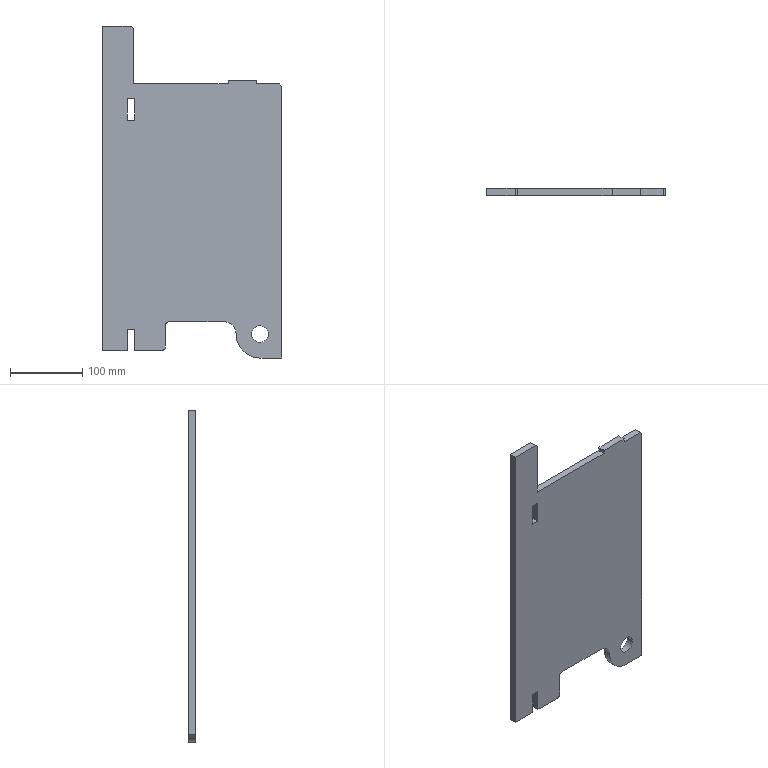Component | SolidWorks | RearUprightPlate-1 | 1 solid | 34 faces | box 247.5 x 10 x 458 mm | volume 902265 mm3 | plane 27 | cylinder 7 | commonest cylinder face diameters 23.2 x2 33.314 x2 10 x2 66 x1 | material Q235
build123d program:
from build123d import *

# Parameters (mm, degrees)
SKETCH1_R           = 11.6
BOSS_EXTRUDE1_DEPTH = 10


with BuildPart() as part:
    # Sketch1 → Boss-Extrude1 (new body)
    with BuildSketch(Plane.XY):
        with BuildLine():
            Line((3719.424, 1887.781), (3719.424, 1862.781))
            Line((3719.424, 1862.781), (3719.424, 1857.781))
            ThreePointArc((3719.424, 1857.781), (3720.888, 1854.245), (3724.424, 1852.781))
            Line((3724.424, 1852.781), (3754.824, 1852.781))
            Line((3754.824, 1852.781), (3755.824, 1852.781))
            Line((3755.824, 1852.781), (3758.924, 1852.781))
            Line((3758.924, 1852.781), (3761.824, 1852.781))
            Line((3761.824, 1852.781), (3761.824, 1882.781))
            Line((3761.824, 1882.781), (3772.024, 1882.781))
            Line((3772.024, 1882.781), (3772.024, 1852.781))
            Line((3772.024, 1852.781), (3774.824, 1852.781))
            Line((3774.824, 1852.781), (3806.424, 1852.781))
            Line((3806.424, 1852.781), (3806.424, 2300.781))
            Line((3806.424, 2300.781), (3766.424, 2300.781))
            Line((3766.424, 2300.781), (3763.424, 2297.781))
            Line((3763.424, 2297.781), (3763.424, 2250.781))
            Line((3763.424, 2250.781), (3763.424, 2220.781))
            Line((3763.424, 2220.781), (3632.924, 2220.781))
            Line((3632.924, 2220.781), (3632.924, 2225.781))
            Line((3632.924, 2225.781), (3593.924, 2225.781))
            Line((3593.924, 2225.781), (3593.924, 2220.781))
            Line((3593.924, 2220.781), (3561.924, 2220.781))
            Line((3561.924, 2220.781), (3558.924, 2217.781))
            Line((3558.924, 2217.781), (3558.924, 1842.781))
            Line((3558.924, 1842.781), (3577.54, 1842.781))
            Line((3577.54, 1842.781), (3588.924, 1842.781))
            ThreePointArc((3588.924, 1842.781), (3612.258, 1852.446), (3621.924, 1875.781))
            ThreePointArc((3621.924, 1875.781), (3626.519, 1887.627), (3638.131, 1892.787))
            Line((3638.131, 1892.787), (3713.924, 1892.781))
            Line((3713.924, 1892.781), (3714.424, 1892.781))
            ThreePointArc((3714.424, 1892.781), (3717.959, 1891.316), (3719.424, 1887.781))
        make_face()
        with Locations((3588.924, 1875.781)):
            Circle(SKETCH1_R, mode=Mode.SUBTRACT)
        Polygon((3772.024, 2170.781), (3761.824, 2170.781), (3761.824, 2200.781), (3772.024, 2200.781), (3772.024, 2190.781), align=None, mode=Mode.SUBTRACT)
    extrude(amount=BOSS_EXTRUDE1_DEPTH)


solid = part.part

# Placed as in the assembly
solid = solid.moved(Location((3301.77, -165.326, 514.924), (-90, 0, 180)))
STEP:
#1=CARTESIAN_POINT('',(-10.849,-6.115,94.122));
#2=VERTEX_POINT('',#1);
#3=CARTESIAN_POINT('',(-11.762,-6.115,94.122));
#4=VERTEX_POINT('',#3);
#5=CARTESIAN_POINT('',(-11.305,-6.115,94.122));
#6=DIRECTION('',(-0.,1.,-0.));
#7=DIRECTION('',(-1.,0.,0.));
#8=AXIS2_PLACEMENT_3D('',#5,#6,#7);
#9=CIRCLE('',#8,0.4567);
#10=EDGE_CURVE('',#2,#4,#9,.T.);
#11=ORIENTED_EDGE('',*,*,#10,.T.);
#12=CARTESIAN_POINT('',(-11.762,-6.509,94.122));
#13=VERTEX_POINT('',#12);
#14=CARTESIAN_POINT('',(-11.762,-6.115,94.122));
#15=DIRECTION('',(0.,-1.,0.));
#16=VECTOR('',#15,39.37);
#17=LINE('',#14,#16);
#18=EDGE_CURVE('',#4,#13,#17,.T.);
#19=ORIENTED_EDGE('',*,*,#18,.T.);
#20=CARTESIAN_POINT('',(-10.849,-6.509,94.122));
#21=VERTEX_POINT('',#20);
#22=CARTESIAN_POINT('',(-11.305,-6.509,94.122));
#23=DIRECTION('',(-0.,1.,-0.));
#24=DIRECTION('',(-1.,0.,0.));
#25=AXIS2_PLACEMENT_3D('',#22,#23,#24);
#26=CIRCLE('',#25,0.4567);
#27=EDGE_CURVE('',#21,#13,#26,.T.);
#28=ORIENTED_EDGE('',*,*,#27,.F.);
#29=CARTESIAN_POINT('',(-10.849,-6.115,94.122));
#30=DIRECTION('',(0.,-1.,0.));
#31=VECTOR('',#30,39.37);
#32=LINE('',#29,#31);
#33=EDGE_CURVE('',#2,#21,#32,.T.);
#34=ORIENTED_EDGE('',*,*,#33,.F.);
#35=EDGE_LOOP('',(#11,#19,#28,#34));
#36=FACE_OUTER_BOUND('',#35,.T.);
#37=CARTESIAN_POINT('',(-11.305,-6.115,94.122));
#38=DIRECTION('',(0.,-1.,0.));
#39=DIRECTION('',(1.,0.,0.));
#40=AXIS2_PLACEMENT_3D('',#37,#38,#39);
#41=CYLINDRICAL_SURFACE('',#40,0.4567);
#42=ADVANCED_FACE('',(#36),#41,.F.);
#43=CARTESIAN_POINT('',(-13.243,-6.115,94.792));
#44=VERTEX_POINT('',#43);
#45=CARTESIAN_POINT('',(-12.604,-6.115,94.136));
#46=VERTEX_POINT('',#45);
#47=CARTESIAN_POINT('',(-13.26,-6.115,94.136));
#48=DIRECTION('',(-0.,1.,-0.));
#49=DIRECTION('',(-1.,0.,0.));
#50=AXIS2_PLACEMENT_3D('',#47,#48,#49);
#51=CIRCLE('',#50,0.6558);
#52=EDGE_CURVE('',#44,#46,#51,.T.);
#53=ORIENTED_EDGE('',*,*,#52,.T.);
#54=CARTESIAN_POINT('',(-12.604,-6.509,94.136));
#55=VERTEX_POINT('',#54);
#56=CARTESIAN_POINT('',(-12.604,-6.115,94.136));
#57=DIRECTION('',(0.,-1.,0.));
#58=VECTOR('',#57,39.37);
#59=LINE('',#56,#58);
#60=EDGE_CURVE('',#46,#55,#59,.T.);
#61=ORIENTED_EDGE('',*,*,#60,.T.);
#62=CARTESIAN_POINT('',(-13.243,-6.509,94.792));
#63=VERTEX_POINT('',#62);
#64=CARTESIAN_POINT('',(-13.26,-6.509,94.136));
#65=DIRECTION('',(-0.,1.,-0.));
#66=DIRECTION('',(-1.,0.,0.));
#67=AXIS2_PLACEMENT_3D('',#64,#65,#66);
#68=CIRCLE('',#67,0.6558);
#69=EDGE_CURVE('',#63,#55,#68,.T.);
#70=ORIENTED_EDGE('',*,*,#69,.F.);
#71=CARTESIAN_POINT('',(-13.243,-6.115,94.792));
#72=DIRECTION('',(0.,-1.,0.));
#73=VECTOR('',#72,39.37);
#74=LINE('',#71,#73);
#75=EDGE_CURVE('',#44,#63,#74,.T.);
#76=ORIENTED_EDGE('',*,*,#75,.F.);
#77=EDGE_LOOP('',(#53,#61,#70,#76));
#78=FACE_OUTER_BOUND('',#77,.T.);
#79=CARTESIAN_POINT('',(-13.26,-6.115,94.136));
#80=DIRECTION('',(0.,-1.,0.));
#81=DIRECTION('',(1.,0.,0.));
#82=AXIS2_PLACEMENT_3D('',#79,#80,#81);
#83=CYLINDRICAL_SURFACE('',#82,0.6558);
#84=ADVANCED_FACE('',(#78),#83,.F.);
#85=CARTESIAN_POINT('',(-11.305,-6.509,92.823));
#86=VERTEX_POINT('',#85);
#87=CARTESIAN_POINT('',(-10.124,-6.509,92.823));
#88=VERTEX_POINT('',#87);
#89=CARTESIAN_POINT('',(129.991,-6.509,92.823));
#90=DIRECTION('',(1.,0.,0.));
#91=VECTOR('',#90,39.37);
#92=LINE('',#89,#91);
#93=EDGE_CURVE('',#86,#88,#92,.T.);
#94=ORIENTED_EDGE('',*,*,#93,.F.);
#95=CARTESIAN_POINT('',(-11.305,-6.115,92.823));
#96=VERTEX_POINT('',#95);
#97=CARTESIAN_POINT('',(-11.305,-6.115,92.823));
#98=DIRECTION('',(0.,-1.,0.));
#99=VECTOR('',#98,39.37);
#100=LINE('',#97,#99);
#101=EDGE_CURVE('',#96,#86,#100,.T.);
#102=ORIENTED_EDGE('',*,*,#101,.F.);
#103=CARTESIAN_POINT('',(-10.124,-6.115,92.823));
#104=VERTEX_POINT('',#103);
#105=CARTESIAN_POINT('',(129.991,-6.115,92.823));
#106=DIRECTION('',(1.,0.,0.));
#107=VECTOR('',#106,39.37);
#108=LINE('',#105,#107);
#109=EDGE_CURVE('',#96,#104,#108,.T.);
#110=ORIENTED_EDGE('',*,*,#109,.T.);
#111=CARTESIAN_POINT('',(-10.124,-6.115,92.823));
#112=DIRECTION('',(0.,-1.,0.));
#113=VECTOR('',#112,39.37);
#114=LINE('',#111,#113);
#115=EDGE_CURVE('',#104,#88,#114,.T.);
#116=ORIENTED_EDGE('',*,*,#115,.T.);
#117=EDGE_LOOP('',(#94,#102,#110,#116));
#118=FACE_OUTER_BOUND('',#117,.T.);
#119=CARTESIAN_POINT('',(129.991,-6.115,92.823));
#120=DIRECTION('',(0.,-0.,-1.));
#121=DIRECTION('',(0.,-1.,0.));
#122=AXIS2_PLACEMENT_3D('',#119,#120,#121);
#123=PLANE('',#122);
#124=ADVANCED_FACE('',(#118),#123,.T.);
#125=CARTESIAN_POINT('',(-12.604,-6.509,94.122));
#126=VERTEX_POINT('',#125);
#127=CARTESIAN_POINT('',(-11.305,-6.509,94.122));
#128=DIRECTION('',(-0.,1.,-0.));
#129=DIRECTION('',(-1.,0.,0.));
#130=AXIS2_PLACEMENT_3D('',#127,#128,#129);
#131=CIRCLE('',#130,1.299);
#132=EDGE_CURVE('',#86,#126,#131,.T.);
#133=ORIENTED_EDGE('',*,*,#132,.T.);
#134=CARTESIAN_POINT('',(-12.604,-6.115,94.122));
#135=VERTEX_POINT('',#134);
#136=CARTESIAN_POINT('',(-12.604,-6.115,94.122));
#137=DIRECTION('',(0.,-1.,0.));
#138=VECTOR('',#137,39.37);
#139=LINE('',#136,#138);
#140=EDGE_CURVE('',#135,#126,#139,.T.);
#141=ORIENTED_EDGE('',*,*,#140,.F.);
#142=CARTESIAN_POINT('',(-11.305,-6.115,94.122));
#143=DIRECTION('',(-0.,1.,-0.));
#144=DIRECTION('',(-1.,0.,0.));
#145=AXIS2_PLACEMENT_3D('',#142,#143,#144);
#146=CIRCLE('',#145,1.299);
#147=EDGE_CURVE('',#96,#135,#146,.T.);
#148=ORIENTED_EDGE('',*,*,#147,.F.);
#149=ORIENTED_EDGE('',*,*,#101,.T.);
#150=EDGE_LOOP('',(#133,#141,#148,#149));
#151=FACE_OUTER_BOUND('',#150,.T.);
#152=CARTESIAN_POINT('',(-11.305,-6.115,94.122));
#153=DIRECTION('',(0.,-1.,0.));
#154=DIRECTION('',(1.,0.,0.));
#155=AXIS2_PLACEMENT_3D('',#152,#153,#154);
#156=CYLINDRICAL_SURFACE('',#155,1.299);
#157=ADVANCED_FACE('',(#151),#156,.T.);
#158=ORIENTED_EDGE('',*,*,#60,.F.);
#159=CARTESIAN_POINT('',(-13.26,-6.115,94.136));
#160=DIRECTION('',(-0.,1.,-0.));
#161=DIRECTION('',(-1.,0.,0.));
#162=AXIS2_PLACEMENT_3D('',#159,#160,#161);
#163=CIRCLE('',#162,0.6558);
#164=EDGE_CURVE('',#46,#135,#163,.T.);
#165=ORIENTED_EDGE('',*,*,#164,.T.);
#166=ORIENTED_EDGE('',*,*,#140,.T.);
#167=CARTESIAN_POINT('',(-13.26,-6.509,94.136));
#168=DIRECTION('',(-0.,1.,-0.));
#169=DIRECTION('',(-1.,0.,0.));
#170=AXIS2_PLACEMENT_3D('',#167,#168,#169);
#171=CIRCLE('',#170,0.6558);
#172=EDGE_CURVE('',#55,#126,#171,.T.);
#173=ORIENTED_EDGE('',*,*,#172,.F.);
#174=EDGE_LOOP('',(#158,#165,#166,#173));
#175=FACE_OUTER_BOUND('',#174,.T.);
#176=CARTESIAN_POINT('',(-13.26,-6.115,94.136));
#177=DIRECTION('',(0.,-1.,0.));
#178=DIRECTION('',(1.,0.,0.));
#179=AXIS2_PLACEMENT_3D('',#176,#177,#178);
#180=CYLINDRICAL_SURFACE('',#179,0.6558);
#181=ADVANCED_FACE('',(#175),#180,.F.);
#182=CARTESIAN_POINT('',(-16.227,-6.509,94.792));
#183=VERTEX_POINT('',#182);
#184=CARTESIAN_POINT('',(129.985,-6.509,94.803));
#185=DIRECTION('',(-1.,-0.,-0.00008077));
#186=VECTOR('',#185,39.37);
#187=LINE('',#184,#186);
#188=EDGE_CURVE('',#63,#183,#187,.T.);
#189=ORIENTED_EDGE('',*,*,#188,.T.);
#190=CARTESIAN_POINT('',(-16.227,-6.115,94.792));
#191=VERTEX_POINT('',#190);
#192=CARTESIAN_POINT('',(-16.227,-6.115,94.792));
#193=DIRECTION('',(0.,-1.,0.));
#194=VECTOR('',#193,39.37);
#195=LINE('',#192,#194);
#196=EDGE_CURVE('',#191,#183,#195,.T.);
#197=ORIENTED_EDGE('',*,*,#196,.F.);
#198=CARTESIAN_POINT('',(129.985,-6.115,94.803));
#199=DIRECTION('',(-1.,-0.,-0.00008077));
#200=VECTOR('',#199,39.37);
#201=LINE('',#198,#200);
#202=EDGE_CURVE('',#44,#191,#201,.T.);
#203=ORIENTED_EDGE('',*,*,#202,.F.);
#204=ORIENTED_EDGE('',*,*,#75,.T.);
#205=EDGE_LOOP('',(#189,#197,#203,#204));
#206=FACE_OUTER_BOUND('',#205,.T.);
#207=CARTESIAN_POINT('',(129.985,-6.115,94.803));
#208=DIRECTION('',(-0.00008077,0.,1.));
#209=DIRECTION('',(1.,0.,0.00008077));
#210=AXIS2_PLACEMENT_3D('',#207,#208,#209);
#211=PLANE('',#210);
#212=ADVANCED_FACE('',(#206),#211,.F.);
#213=CARTESIAN_POINT('',(-16.246,-6.509,94.792));
#214=VERTEX_POINT('',#213);
#215=CARTESIAN_POINT('',(129.991,-6.509,94.792));
#216=DIRECTION('',(-1.,-0.,-0.));
#217=VECTOR('',#216,39.37);
#218=LINE('',#215,#217);
#219=EDGE_CURVE('',#183,#214,#218,.T.);
#220=ORIENTED_EDGE('',*,*,#219,.T.);
#221=CARTESIAN_POINT('',(-16.246,-6.115,94.792));
#222=VERTEX_POINT('',#221);
#223=CARTESIAN_POINT('',(-16.246,-6.115,94.792));
#224=DIRECTION('',(0.,-1.,0.));
#225=VECTOR('',#224,39.37);
#226=LINE('',#223,#225);
#227=EDGE_CURVE('',#222,#214,#226,.T.);
#228=ORIENTED_EDGE('',*,*,#227,.F.);
#229=CARTESIAN_POINT('',(129.991,-6.115,94.792));
#230=DIRECTION('',(-1.,-0.,-0.));
#231=VECTOR('',#230,39.37);
#232=LINE('',#229,#231);
#233=EDGE_CURVE('',#191,#222,#232,.T.);
#234=ORIENTED_EDGE('',*,*,#233,.F.);
#235=ORIENTED_EDGE('',*,*,#196,.T.);
#236=EDGE_LOOP('',(#220,#228,#234,#235));
#237=FACE_OUTER_BOUND('',#236,.T.);
#238=CARTESIAN_POINT('',(129.991,-6.115,94.792));
#239=DIRECTION('',(-0.,0.,1.));
#240=DIRECTION('',(-0.,1.,-0.));
#241=AXIS2_PLACEMENT_3D('',#238,#239,#240);
#242=PLANE('',#241);
#243=ADVANCED_FACE('',(#237),#242,.F.);
#244=CARTESIAN_POINT('',(-16.443,-6.509,94.595));
#245=VERTEX_POINT('',#244);
#246=CARTESIAN_POINT('',(-16.246,-6.509,94.595));
#247=DIRECTION('',(-0.,1.,-0.));
#248=DIRECTION('',(-1.,0.,0.));
#249=AXIS2_PLACEMENT_3D('',#246,#247,#248);
#250=CIRCLE('',#249,0.1969);
#251=EDGE_CURVE('',#245,#214,#250,.T.);
#252=ORIENTED_EDGE('',*,*,#251,.F.);
#253=CARTESIAN_POINT('',(-16.443,-6.115,94.595));
#254=VERTEX_POINT('',#253);
#255=CARTESIAN_POINT('',(-16.443,-6.115,94.595));
#256=DIRECTION('',(0.,-1.,0.));
#257=VECTOR('',#256,39.37);
#258=LINE('',#255,#257);
#259=EDGE_CURVE('',#254,#245,#258,.T.);
#260=ORIENTED_EDGE('',*,*,#259,.F.);
#261=CARTESIAN_POINT('',(-16.246,-6.115,94.595));
#262=DIRECTION('',(-0.,1.,-0.));
#263=DIRECTION('',(-1.,0.,0.));
#264=AXIS2_PLACEMENT_3D('',#261,#262,#263);
#265=CIRCLE('',#264,0.1969);
#266=EDGE_CURVE('',#254,#222,#265,.T.);
#267=ORIENTED_EDGE('',*,*,#266,.T.);
#268=ORIENTED_EDGE('',*,*,#227,.T.);
#269=EDGE_LOOP('',(#252,#260,#267,#268));
#270=FACE_OUTER_BOUND('',#269,.T.);
#271=CARTESIAN_POINT('',(-16.246,-6.115,94.595));
#272=DIRECTION('',(0.,-1.,0.));
#273=DIRECTION('',(1.,0.,0.));
#274=AXIS2_PLACEMENT_3D('',#271,#272,#273);
#275=CYLINDRICAL_SURFACE('',#274,0.1969);
#276=ADVANCED_FACE('',(#270),#275,.F.);
#277=CARTESIAN_POINT('',(-16.443,-6.509,93.61));
#278=VERTEX_POINT('',#277);
#279=CARTESIAN_POINT('',(-16.443,-6.509,20.273));
#280=DIRECTION('',(-0.00000029,0.,1.));
#281=VECTOR('',#280,39.37);
#282=LINE('',#279,#281);
#283=EDGE_CURVE('',#278,#245,#282,.T.);
#284=ORIENTED_EDGE('',*,*,#283,.F.);
#285=CARTESIAN_POINT('',(-16.443,-6.115,93.61));
#286=VERTEX_POINT('',#285);
#287=CARTESIAN_POINT('',(-16.443,-6.115,93.61));
#288=DIRECTION('',(0.,-1.,0.));
#289=VECTOR('',#288,39.37);
#290=LINE('',#287,#289);
#291=EDGE_CURVE('',#286,#278,#290,.T.);
#292=ORIENTED_EDGE('',*,*,#291,.F.);
#293=CARTESIAN_POINT('',(-16.443,-6.115,20.273));
#294=DIRECTION('',(-0.00000029,0.,1.));
#295=VECTOR('',#294,39.37);
#296=LINE('',#293,#295);
#297=EDGE_CURVE('',#286,#254,#296,.T.);
#298=ORIENTED_EDGE('',*,*,#297,.T.);
#299=ORIENTED_EDGE('',*,*,#259,.T.);
#300=EDGE_LOOP('',(#284,#292,#298,#299));
#301=FACE_OUTER_BOUND('',#300,.T.);
#302=CARTESIAN_POINT('',(-16.443,-6.115,20.273));
#303=DIRECTION('',(1.,0.,0.00000029));
#304=DIRECTION('',(0.00000029,-0.,-1.));
#305=AXIS2_PLACEMENT_3D('',#302,#303,#304);
#306=PLANE('',#305);
#307=ADVANCED_FACE('',(#301),#306,.T.);
#308=CARTESIAN_POINT('',(-16.443,-6.509,93.414));
#309=VERTEX_POINT('',#308);
#310=CARTESIAN_POINT('',(-16.443,-6.509,20.273));
#311=DIRECTION('',(-0.00000143,-0.,-1.));
#312=VECTOR('',#311,39.37);
#313=LINE('',#310,#312);
#314=EDGE_CURVE('',#278,#309,#313,.T.);
#315=ORIENTED_EDGE('',*,*,#314,.T.);
#316=CARTESIAN_POINT('',(-16.443,-6.115,93.414));
#317=VERTEX_POINT('',#316);
#318=CARTESIAN_POINT('',(-16.443,-6.115,93.414));
#319=DIRECTION('',(0.,-1.,0.));
#320=VECTOR('',#319,39.37);
#321=LINE('',#318,#320);
#322=EDGE_CURVE('',#317,#309,#321,.T.);
#323=ORIENTED_EDGE('',*,*,#322,.F.);
#324=CARTESIAN_POINT('',(-16.443,-6.115,20.273));
#325=DIRECTION('',(-0.00000143,-0.,-1.));
#326=VECTOR('',#325,39.37);
#327=LINE('',#324,#326);
#328=EDGE_CURVE('',#286,#317,#327,.T.);
#329=ORIENTED_EDGE('',*,*,#328,.F.);
#330=ORIENTED_EDGE('',*,*,#291,.T.);
#331=EDGE_LOOP('',(#315,#323,#329,#330));
#332=FACE_OUTER_BOUND('',#331,.T.);
#333=CARTESIAN_POINT('',(-16.443,-6.115,20.273));
#334=DIRECTION('',(-1.,-0.,0.00000143));
#335=DIRECTION('',(0.00000143,0.,1.));
#336=AXIS2_PLACEMENT_3D('',#333,#334,#335);
#337=PLANE('',#336);
#338=ADVANCED_FACE('',(#332),#337,.F.);
#339=CARTESIAN_POINT('',(-16.64,-6.509,93.217));
#340=VERTEX_POINT('',#339);
#341=CARTESIAN_POINT('',(-16.64,-6.509,93.414));
#342=DIRECTION('',(-0.,1.,-0.));
#343=DIRECTION('',(-1.,0.,0.));
#344=AXIS2_PLACEMENT_3D('',#341,#342,#343);
#345=CIRCLE('',#344,0.1969);
#346=EDGE_CURVE('',#309,#340,#345,.T.);
#347=ORIENTED_EDGE('',*,*,#346,.T.);
#348=CARTESIAN_POINT('',(-16.64,-6.115,93.217));
#349=VERTEX_POINT('',#348);
#350=CARTESIAN_POINT('',(-16.64,-6.115,93.217));
#351=DIRECTION('',(0.,-1.,0.));
#352=VECTOR('',#351,39.37);
#353=LINE('',#350,#352);
#354=EDGE_CURVE('',#349,#340,#353,.T.);
#355=ORIENTED_EDGE('',*,*,#354,.F.);
#356=CARTESIAN_POINT('',(-16.64,-6.115,93.414));
#357=DIRECTION('',(-0.,1.,-0.));
#358=DIRECTION('',(-1.,0.,0.));
#359=AXIS2_PLACEMENT_3D('',#356,#357,#358);
#360=CIRCLE('',#359,0.1969);
#361=EDGE_CURVE('',#317,#349,#360,.T.);
#362=ORIENTED_EDGE('',*,*,#361,.F.);
#363=ORIENTED_EDGE('',*,*,#322,.T.);
#364=EDGE_LOOP('',(#347,#355,#362,#363));
#365=FACE_OUTER_BOUND('',#364,.T.);
#366=CARTESIAN_POINT('',(-16.64,-6.115,93.414));
#367=DIRECTION('',(0.,-1.,0.));
#368=DIRECTION('',(1.,0.,0.));
#369=AXIS2_PLACEMENT_3D('',#366,#367,#368);
#370=CYLINDRICAL_SURFACE('',#369,0.1969);
#371=ADVANCED_FACE('',(#365),#370,.T.);
#372=CARTESIAN_POINT('',(-18.112,-6.509,93.217));
#373=VERTEX_POINT('',#372);
#374=CARTESIAN_POINT('',(129.991,-6.509,93.217));
#375=DIRECTION('',(-1.,-0.,-0.));
#376=VECTOR('',#375,39.37);
#377=LINE('',#374,#376);
#378=EDGE_CURVE('',#340,#373,#377,.T.);
#379=ORIENTED_EDGE('',*,*,#378,.T.);
#380=CARTESIAN_POINT('',(-18.112,-6.115,93.217));
#381=VERTEX_POINT('',#380);
#382=CARTESIAN_POINT('',(-18.112,-6.115,93.217));
#383=DIRECTION('',(0.,-1.,0.));
#384=VECTOR('',#383,39.37);
#385=LINE('',#382,#384);
#386=EDGE_CURVE('',#381,#373,#385,.T.);
#387=ORIENTED_EDGE('',*,*,#386,.F.);
#388=CARTESIAN_POINT('',(129.991,-6.115,93.217));
#389=DIRECTION('',(-1.,-0.,-0.));
#390=VECTOR('',#389,39.37);
#391=LINE('',#388,#390);
#392=EDGE_CURVE('',#349,#381,#391,.T.);
#393=ORIENTED_EDGE('',*,*,#392,.F.);
#394=ORIENTED_EDGE('',*,*,#354,.T.);
#395=EDGE_LOOP('',(#379,#387,#393,#394));
#396=FACE_OUTER_BOUND('',#395,.T.);
#397=CARTESIAN_POINT('',(129.991,-6.115,93.217));
#398=DIRECTION('',(-0.,0.,1.));
#399=DIRECTION('',(-0.,1.,-0.));
#400=AXIS2_PLACEMENT_3D('',#397,#398,#399);
#401=PLANE('',#400);
#402=ADVANCED_FACE('',(#396),#401,.F.);
#403=CARTESIAN_POINT('',(-18.112,-6.509,94.398));
#404=VERTEX_POINT('',#403);
#405=CARTESIAN_POINT('',(-18.112,-6.509,20.273));
#406=DIRECTION('',(-0.,0.,1.));
#407=VECTOR('',#406,39.37);
#408=LINE('',#405,#407);
#409=EDGE_CURVE('',#373,#404,#408,.T.);
#410=ORIENTED_EDGE('',*,*,#409,.T.);
#411=CARTESIAN_POINT('',(-18.112,-6.115,94.398));
#412=VERTEX_POINT('',#411);
#413=CARTESIAN_POINT('',(-18.112,-6.115,94.398));
#414=DIRECTION('',(0.,-1.,0.));
#415=VECTOR('',#414,39.37);
#416=LINE('',#413,#415);
#417=EDGE_CURVE('',#412,#404,#416,.T.);
#418=ORIENTED_EDGE('',*,*,#417,.F.);
#419=CARTESIAN_POINT('',(-18.112,-6.115,20.273));
#420=DIRECTION('',(-0.,0.,1.));
#421=VECTOR('',#420,39.37);
#422=LINE('',#419,#421);
#423=EDGE_CURVE('',#381,#412,#422,.T.);
#424=ORIENTED_EDGE('',*,*,#423,.F.);
#425=ORIENTED_EDGE('',*,*,#386,.T.);
#426=EDGE_LOOP('',(#410,#418,#424,#425));
#427=FACE_OUTER_BOUND('',#426,.T.);
#428=CARTESIAN_POINT('',(-18.112,-6.115,20.273));
#429=DIRECTION('',(1.,0.,0.));
#430=DIRECTION('',(-0.,1.,-0.));
#431=AXIS2_PLACEMENT_3D('',#428,#429,#430);
#432=PLANE('',#431);
#433=ADVANCED_FACE('',(#427),#432,.F.);
#434=CARTESIAN_POINT('',(-18.514,-6.509,94.398));
#435=VERTEX_POINT('',#434);
#436=CARTESIAN_POINT('',(129.991,-6.509,94.398));
#437=DIRECTION('',(-1.,-0.,-0.));
#438=VECTOR('',#437,39.37);
#439=LINE('',#436,#438);
#440=EDGE_CURVE('',#404,#435,#439,.T.);
#441=ORIENTED_EDGE('',*,*,#440,.T.);
#442=CARTESIAN_POINT('',(-18.514,-6.115,94.398));
#443=VERTEX_POINT('',#442);
#444=CARTESIAN_POINT('',(-18.514,-6.115,94.398));
#445=DIRECTION('',(0.,-1.,0.));
#446=VECTOR('',#445,39.37);
#447=LINE('',#444,#446);
#448=EDGE_CURVE('',#443,#435,#447,.T.);
#449=ORIENTED_EDGE('',*,*,#448,.F.);
#450=CARTESIAN_POINT('',(129.991,-6.115,94.398));
#451=DIRECTION('',(-1.,-0.,-0.));
#452=VECTOR('',#451,39.37);
#453=LINE('',#450,#452);
#454=EDGE_CURVE('',#412,#443,#453,.T.);
#455=ORIENTED_EDGE('',*,*,#454,.F.);
#456=ORIENTED_EDGE('',*,*,#417,.T.);
#457=EDGE_LOOP('',(#441,#449,#455,#456));
#458=FACE_OUTER_BOUND('',#457,.T.);
#459=CARTESIAN_POINT('',(129.991,-6.115,94.398));
#460=DIRECTION('',(-0.,0.,1.));
#461=DIRECTION('',(1.,0.,0.));
#462=AXIS2_PLACEMENT_3D('',#459,#460,#461);
#463=PLANE('',#462);
#464=ADVANCED_FACE('',(#458),#463,.F.);
#465=CARTESIAN_POINT('',(-18.514,-6.509,93.217));
#466=VERTEX_POINT('',#465);
#467=CARTESIAN_POINT('',(-18.514,-6.509,20.273));
#468=DIRECTION('',(0.,-0.,-1.));
#469=VECTOR('',#468,39.37);
#470=LINE('',#467,#469);
#471=EDGE_CURVE('',#435,#466,#470,.T.);
#472=ORIENTED_EDGE('',*,*,#471,.T.);
#473=CARTESIAN_POINT('',(-18.514,-6.115,93.217));
#474=VERTEX_POINT('',#473);
#475=CARTESIAN_POINT('',(-18.514,-6.115,93.217));
#476=DIRECTION('',(0.,-1.,0.));
#477=VECTOR('',#476,39.37);
#478=LINE('',#475,#477);
#479=EDGE_CURVE('',#474,#466,#478,.T.);
#480=ORIENTED_EDGE('',*,*,#479,.F.);
#481=CARTESIAN_POINT('',(-18.514,-6.115,20.273));
#482=DIRECTION('',(0.,-0.,-1.));
#483=VECTOR('',#482,39.37);
#484=LINE('',#481,#483);
#485=EDGE_CURVE('',#443,#474,#484,.T.);
#486=ORIENTED_EDGE('',*,*,#485,.F.);
#487=ORIENTED_EDGE('',*,*,#448,.T.);
#488=EDGE_LOOP('',(#472,#480,#486,#487));
#489=FACE_OUTER_BOUND('',#488,.T.);
#490=CARTESIAN_POINT('',(-18.514,-6.115,20.273));
#491=DIRECTION('',(-1.,-0.,-0.));
#492=DIRECTION('',(0.,-1.,0.));
#493=AXIS2_PLACEMENT_3D('',#490,#491,#492);
#494=PLANE('',#493);
#495=ADVANCED_FACE('',(#489),#494,.F.);
#496=CARTESIAN_POINT('',(-19.868,-6.509,93.217));
#497=VERTEX_POINT('',#496);
#498=CARTESIAN_POINT('',(129.991,-6.509,93.217));
#499=DIRECTION('',(-1.,-0.,-0.));
#500=VECTOR('',#499,39.37);
#501=LINE('',#498,#500);
#502=EDGE_CURVE('',#466,#497,#501,.T.);
#503=ORIENTED_EDGE('',*,*,#502,.T.);
#504=CARTESIAN_POINT('',(-19.868,-6.115,93.217));
#505=VERTEX_POINT('',#504);
#506=CARTESIAN_POINT('',(-19.868,-6.115,93.217));
#507=DIRECTION('',(0.,-1.,0.));
#508=VECTOR('',#507,39.37);
#509=LINE('',#506,#508);
#510=EDGE_CURVE('',#505,#497,#509,.T.);
#511=ORIENTED_EDGE('',*,*,#510,.F.);
#512=CARTESIAN_POINT('',(129.991,-6.115,93.217));
#513=DIRECTION('',(-1.,-0.,-0.));
#514=VECTOR('',#513,39.37);
#515=LINE('',#512,#514);
#516=EDGE_CURVE('',#474,#505,#515,.T.);
#517=ORIENTED_EDGE('',*,*,#516,.F.);
#518=ORIENTED_EDGE('',*,*,#479,.T.);
#519=EDGE_LOOP('',(#503,#511,#517,#518));
#520=FACE_OUTER_BOUND('',#519,.T.);
#521=CARTESIAN_POINT('',(129.991,-6.115,93.217));
#522=DIRECTION('',(-0.,0.,1.));
#523=DIRECTION('',(-0.,1.,-0.));
#524=AXIS2_PLACEMENT_3D('',#521,#522,#523);
#525=PLANE('',#524);
#526=ADVANCED_FACE('',(#520),#525,.F.);
#527=CARTESIAN_POINT('',(-19.868,-6.509,110.855));
#528=VERTEX_POINT('',#527);
#529=CARTESIAN_POINT('',(-19.868,-6.509,20.273));
#530=DIRECTION('',(0.,-0.,-1.));
#531=VECTOR('',#530,39.37);
#532=LINE('',#529,#531);
#533=EDGE_CURVE('',#528,#497,#532,.T.);
#534=ORIENTED_EDGE('',*,*,#533,.F.);
#535=CARTESIAN_POINT('',(-19.868,-6.115,110.855));
#536=VERTEX_POINT('',#535);
#537=CARTESIAN_POINT('',(-19.868,-6.115,110.855));
#538=DIRECTION('',(0.,-1.,0.));
#539=VECTOR('',#538,39.37);
#540=LINE('',#537,#539);
#541=EDGE_CURVE('',#536,#528,#540,.T.);
#542=ORIENTED_EDGE('',*,*,#541,.F.);
#543=CARTESIAN_POINT('',(-19.868,-6.115,20.273));
#544=DIRECTION('',(0.,-0.,-1.));
#545=VECTOR('',#544,39.37);
#546=LINE('',#543,#545);
#547=EDGE_CURVE('',#536,#505,#546,.T.);
#548=ORIENTED_EDGE('',*,*,#547,.T.);
#549=ORIENTED_EDGE('',*,*,#510,.T.);
#550=EDGE_LOOP('',(#534,#542,#548,#549));
#551=FACE_OUTER_BOUND('',#550,.T.);
#552=CARTESIAN_POINT('',(-19.868,-6.115,20.273));
#553=DIRECTION('',(-1.,-0.,-0.));
#554=DIRECTION('',(0.,-1.,0.));
#555=AXIS2_PLACEMENT_3D('',#552,#553,#554);
#556=PLANE('',#555);
#557=ADVANCED_FACE('',(#551),#556,.T.);
#558=CARTESIAN_POINT('',(-18.293,-6.509,110.855));
#559=VERTEX_POINT('',#558);
#560=CARTESIAN_POINT('',(129.991,-6.509,110.855));
#561=DIRECTION('',(-1.,-0.,-0.));
#562=VECTOR('',#561,39.37);
#563=LINE('',#560,#562);
#564=EDGE_CURVE('',#559,#528,#563,.T.);
#565=ORIENTED_EDGE('',*,*,#564,.F.);
#566=CARTESIAN_POINT('',(-18.293,-6.115,110.855));
#567=VERTEX_POINT('',#566);
#568=CARTESIAN_POINT('',(-18.293,-6.115,110.855));
#569=DIRECTION('',(0.,-1.,0.));
#570=VECTOR('',#569,39.37);
#571=LINE('',#568,#570);
#572=EDGE_CURVE('',#567,#559,#571,.T.);
#573=ORIENTED_EDGE('',*,*,#572,.F.);
#574=CARTESIAN_POINT('',(129.991,-6.115,110.855));
#575=DIRECTION('',(-1.,-0.,-0.));
#576=VECTOR('',#575,39.37);
#577=LINE('',#574,#576);
#578=EDGE_CURVE('',#567,#536,#577,.T.);
#579=ORIENTED_EDGE('',*,*,#578,.T.);
#580=ORIENTED_EDGE('',*,*,#541,.T.);
#581=EDGE_LOOP('',(#565,#573,#579,#580));
#582=FACE_OUTER_BOUND('',#581,.T.);
#583=CARTESIAN_POINT('',(129.991,-6.115,110.855));
#584=DIRECTION('',(-0.,0.,1.));
#585=DIRECTION('',(-0.,1.,-0.));
#586=AXIS2_PLACEMENT_3D('',#583,#584,#585);
#587=PLANE('',#586);
#588=ADVANCED_FACE('',(#582),#587,.T.);
#589=CARTESIAN_POINT('',(-18.175,-6.509,110.736));
#590=VERTEX_POINT('',#589);
#591=CARTESIAN_POINT('',(101.14,-6.509,-8.579));
#592=DIRECTION('',(0.7071,0.,-0.7071));
#593=VECTOR('',#592,39.37);
#594=LINE('',#591,#593);
#595=EDGE_CURVE('',#559,#590,#594,.T.);
#596=ORIENTED_EDGE('',*,*,#595,.T.);
#597=CARTESIAN_POINT('',(-18.175,-6.115,110.736));
#598=VERTEX_POINT('',#597);
#599=CARTESIAN_POINT('',(-18.175,-6.115,110.736));
#600=DIRECTION('',(0.,-1.,0.));
#601=VECTOR('',#600,39.37);
#602=LINE('',#599,#601);
#603=EDGE_CURVE('',#598,#590,#602,.T.);
#604=ORIENTED_EDGE('',*,*,#603,.F.);
#605=CARTESIAN_POINT('',(101.14,-6.115,-8.579));
#606=DIRECTION('',(0.7071,0.,-0.7071));
#607=VECTOR('',#606,39.37);
#608=LINE('',#605,#607);
#609=EDGE_CURVE('',#567,#598,#608,.T.);
#610=ORIENTED_EDGE('',*,*,#609,.F.);
#611=ORIENTED_EDGE('',*,*,#572,.T.);
#612=EDGE_LOOP('',(#596,#604,#610,#611));
#613=FACE_OUTER_BOUND('',#612,.T.);
#614=CARTESIAN_POINT('',(101.14,-6.115,-8.579));
#615=DIRECTION('',(-0.7071,-0.,-0.7071));
#616=DIRECTION('',(-0.7071,-0.,0.7071));
#617=AXIS2_PLACEMENT_3D('',#614,#615,#616);
#618=PLANE('',#617);
#619=ADVANCED_FACE('',(#613),#618,.F.);
#620=CARTESIAN_POINT('',(-18.175,-6.509,107.705));
#621=VERTEX_POINT('',#620);
#622=CARTESIAN_POINT('',(-18.175,-6.509,20.273));
#623=DIRECTION('',(-0.,0.,1.));
#624=VECTOR('',#623,39.37);
#625=LINE('',#622,#624);
#626=EDGE_CURVE('',#621,#590,#625,.T.);
#627=ORIENTED_EDGE('',*,*,#626,.F.);
#628=CARTESIAN_POINT('',(-18.175,-6.115,107.705));
#629=VERTEX_POINT('',#628);
#630=CARTESIAN_POINT('',(-18.175,-6.115,107.705));
#631=DIRECTION('',(0.,-1.,0.));
#632=VECTOR('',#631,39.37);
#633=LINE('',#630,#632);
#634=EDGE_CURVE('',#629,#621,#633,.T.);
#635=ORIENTED_EDGE('',*,*,#634,.F.);
#636=CARTESIAN_POINT('',(-18.175,-6.115,20.273));
#637=DIRECTION('',(-0.,0.,1.));
#638=VECTOR('',#637,39.37);
#639=LINE('',#636,#638);
#640=EDGE_CURVE('',#629,#598,#639,.T.);
#641=ORIENTED_EDGE('',*,*,#640,.T.);
#642=ORIENTED_EDGE('',*,*,#603,.T.);
#643=EDGE_LOOP('',(#627,#635,#641,#642));
#644=FACE_OUTER_BOUND('',#643,.T.);
#645=CARTESIAN_POINT('',(-18.175,-6.115,20.273));
#646=DIRECTION('',(1.,0.,0.));
#647=DIRECTION('',(-0.,1.,-0.));
#648=AXIS2_PLACEMENT_3D('',#645,#646,#647);
#649=PLANE('',#648);
#650=ADVANCED_FACE('',(#644),#649,.T.);
#651=CARTESIAN_POINT('',(-13.038,-6.509,107.705));
#652=VERTEX_POINT('',#651);
#653=CARTESIAN_POINT('',(129.991,-6.509,107.705));
#654=DIRECTION('',(-1.,-0.,-0.));
#655=VECTOR('',#654,39.37);
#656=LINE('',#653,#655);
#657=EDGE_CURVE('',#652,#621,#656,.T.);
#658=ORIENTED_EDGE('',*,*,#657,.F.);
#659=CARTESIAN_POINT('',(-13.038,-6.115,107.705));
#660=VERTEX_POINT('',#659);
#661=CARTESIAN_POINT('',(-13.038,-6.115,107.705));
#662=DIRECTION('',(0.,-1.,0.));
#663=VECTOR('',#662,39.37);
#664=LINE('',#661,#663);
#665=EDGE_CURVE('',#660,#652,#664,.T.);
#666=ORIENTED_EDGE('',*,*,#665,.F.);
#667=CARTESIAN_POINT('',(129.991,-6.115,107.705));
#668=DIRECTION('',(-1.,-0.,-0.));
#669=VECTOR('',#668,39.37);
#670=LINE('',#667,#669);
#671=EDGE_CURVE('',#660,#629,#670,.T.);
#672=ORIENTED_EDGE('',*,*,#671,.T.);
#673=ORIENTED_EDGE('',*,*,#634,.T.);
#674=EDGE_LOOP('',(#658,#666,#672,#673));
#675=FACE_OUTER_BOUND('',#674,.T.);
#676=CARTESIAN_POINT('',(129.991,-6.115,107.705));
#677=DIRECTION('',(-0.,0.,1.));
#678=DIRECTION('',(-0.,1.,-0.));
#679=AXIS2_PLACEMENT_3D('',#676,#677,#678);
#680=PLANE('',#679);
#681=ADVANCED_FACE('',(#675),#680,.T.);
#682=CARTESIAN_POINT('',(-13.038,-6.509,107.902));
#683=VERTEX_POINT('',#682);
#684=CARTESIAN_POINT('',(-13.038,-6.509,20.273));
#685=DIRECTION('',(0.,-0.,-1.));
#686=VECTOR('',#685,39.37);
#687=LINE('',#684,#686);
#688=EDGE_CURVE('',#683,#652,#687,.T.);
#689=ORIENTED_EDGE('',*,*,#688,.F.);
#690=CARTESIAN_POINT('',(-13.038,-6.115,107.902));
#691=VERTEX_POINT('',#690);
#692=CARTESIAN_POINT('',(-13.038,-6.115,107.902));
#693=DIRECTION('',(0.,-1.,0.));
#694=VECTOR('',#693,39.37);
#695=LINE('',#692,#694);
#696=EDGE_CURVE('',#691,#683,#695,.T.);
#697=ORIENTED_EDGE('',*,*,#696,.F.);
#698=CARTESIAN_POINT('',(-13.038,-6.115,20.273));
#699=DIRECTION('',(0.,-0.,-1.));
#700=VECTOR('',#699,39.37);
#701=LINE('',#698,#700);
#702=EDGE_CURVE('',#691,#660,#701,.T.);
#703=ORIENTED_EDGE('',*,*,#702,.T.);
#704=ORIENTED_EDGE('',*,*,#665,.T.);
#705=EDGE_LOOP('',(#689,#697,#703,#704));
#706=FACE_OUTER_BOUND('',#705,.T.);
#707=CARTESIAN_POINT('',(-13.038,-6.115,20.273));
#708=DIRECTION('',(-1.,-0.,-0.));
#709=DIRECTION('',(0.,-1.,0.));
#710=AXIS2_PLACEMENT_3D('',#707,#708,#709);
#711=PLANE('',#710);
#712=ADVANCED_FACE('',(#706),#711,.T.);
#713=CARTESIAN_POINT('',(-11.502,-6.509,107.902));
#714=VERTEX_POINT('',#713);
#715=CARTESIAN_POINT('',(129.991,-6.509,107.902));
#716=DIRECTION('',(-1.,-0.,-0.));
#717=VECTOR('',#716,39.37);
#718=LINE('',#715,#717);
#719=EDGE_CURVE('',#714,#683,#718,.T.);
#720=ORIENTED_EDGE('',*,*,#719,.F.);
#721=CARTESIAN_POINT('',(-11.502,-6.115,107.902));
#722=VERTEX_POINT('',#721);
#723=CARTESIAN_POINT('',(-11.502,-6.115,107.902));
#724=DIRECTION('',(0.,-1.,0.));
#725=VECTOR('',#724,39.37);
#726=LINE('',#723,#725);
#727=EDGE_CURVE('',#722,#714,#726,.T.);
#728=ORIENTED_EDGE('',*,*,#727,.F.);
#729=CARTESIAN_POINT('',(129.991,-6.115,107.902));
#730=DIRECTION('',(-1.,-0.,-0.));
#731=VECTOR('',#730,39.37);
#732=LINE('',#729,#731);
#733=EDGE_CURVE('',#722,#691,#732,.T.);
#734=ORIENTED_EDGE('',*,*,#733,.T.);
#735=ORIENTED_EDGE('',*,*,#696,.T.);
#736=EDGE_LOOP('',(#720,#728,#734,#735));
#737=FACE_OUTER_BOUND('',#736,.T.);
#738=CARTESIAN_POINT('',(129.991,-6.115,107.902));
#739=DIRECTION('',(-0.,0.,1.));
#740=DIRECTION('',(-0.,1.,-0.));
#741=AXIS2_PLACEMENT_3D('',#738,#739,#740);
#742=PLANE('',#741);
#743=ADVANCED_FACE('',(#737),#742,.T.);
#744=CARTESIAN_POINT('',(-11.502,-6.509,107.705));
#745=VERTEX_POINT('',#744);
#746=CARTESIAN_POINT('',(-11.502,-6.509,20.273));
#747=DIRECTION('',(-0.,0.,1.));
#748=VECTOR('',#747,39.37);
#749=LINE('',#746,#748);
#750=EDGE_CURVE('',#745,#714,#749,.T.);
#751=ORIENTED_EDGE('',*,*,#750,.F.);
#752=CARTESIAN_POINT('',(-11.502,-6.115,107.705));
#753=VERTEX_POINT('',#752);
#754=CARTESIAN_POINT('',(-11.502,-6.115,107.705));
#755=DIRECTION('',(0.,-1.,0.));
#756=VECTOR('',#755,39.37);
#757=LINE('',#754,#756);
#758=EDGE_CURVE('',#753,#745,#757,.T.);
#759=ORIENTED_EDGE('',*,*,#758,.F.);
#760=CARTESIAN_POINT('',(-11.502,-6.115,20.273));
#761=DIRECTION('',(-0.,0.,1.));
#762=VECTOR('',#761,39.37);
#763=LINE('',#760,#762);
#764=EDGE_CURVE('',#753,#722,#763,.T.);
#765=ORIENTED_EDGE('',*,*,#764,.T.);
#766=ORIENTED_EDGE('',*,*,#727,.T.);
#767=EDGE_LOOP('',(#751,#759,#765,#766));
#768=FACE_OUTER_BOUND('',#767,.T.);
#769=CARTESIAN_POINT('',(-11.502,-6.115,20.273));
#770=DIRECTION('',(1.,0.,0.));
#771=DIRECTION('',(-0.,1.,-0.));
#772=AXIS2_PLACEMENT_3D('',#769,#770,#771);
#773=PLANE('',#772);
#774=ADVANCED_FACE('',(#768),#773,.T.);
#775=CARTESIAN_POINT('',(-10.242,-6.509,107.705));
#776=VERTEX_POINT('',#775);
#777=CARTESIAN_POINT('',(129.991,-6.509,107.705));
#778=DIRECTION('',(-1.,-0.,-0.));
#779=VECTOR('',#778,39.37);
#780=LINE('',#777,#779);
#781=EDGE_CURVE('',#776,#745,#780,.T.);
#782=ORIENTED_EDGE('',*,*,#781,.F.);
#783=CARTESIAN_POINT('',(-10.242,-6.115,107.705));
#784=VERTEX_POINT('',#783);
#785=CARTESIAN_POINT('',(-10.242,-6.115,107.705));
#786=DIRECTION('',(0.,-1.,0.));
#787=VECTOR('',#786,39.37);
#788=LINE('',#785,#787);
#789=EDGE_CURVE('',#784,#776,#788,.T.);
#790=ORIENTED_EDGE('',*,*,#789,.F.);
#791=CARTESIAN_POINT('',(129.991,-6.115,107.705));
#792=DIRECTION('',(-1.,-0.,-0.));
#793=VECTOR('',#792,39.37);
#794=LINE('',#791,#793);
#795=EDGE_CURVE('',#784,#753,#794,.T.);
#796=ORIENTED_EDGE('',*,*,#795,.T.);
#797=ORIENTED_EDGE('',*,*,#758,.T.);
#798=EDGE_LOOP('',(#782,#790,#796,#797));
#799=FACE_OUTER_BOUND('',#798,.T.);
#800=CARTESIAN_POINT('',(129.991,-6.115,107.705));
#801=DIRECTION('',(-0.,0.,1.));
#802=DIRECTION('',(-0.,1.,-0.));
#803=AXIS2_PLACEMENT_3D('',#800,#801,#802);
#804=PLANE('',#803);
#805=ADVANCED_FACE('',(#799),#804,.T.);
#806=CARTESIAN_POINT('',(-10.124,-6.509,107.587));
#807=VERTEX_POINT('',#806);
#808=CARTESIAN_POINT('',(103.59,-6.509,-6.128));
#809=DIRECTION('',(-0.7071,-0.,0.7071));
#810=VECTOR('',#809,39.37);
#811=LINE('',#808,#810);
#812=EDGE_CURVE('',#807,#776,#811,.T.);
#813=ORIENTED_EDGE('',*,*,#812,.F.);
#814=CARTESIAN_POINT('',(-10.124,-6.115,107.587));
#815=VERTEX_POINT('',#814);
#816=CARTESIAN_POINT('',(-10.124,-6.115,107.587));
#817=DIRECTION('',(0.,-1.,0.));
#818=VECTOR('',#817,39.37);
#819=LINE('',#816,#818);
#820=EDGE_CURVE('',#815,#807,#819,.T.);
#821=ORIENTED_EDGE('',*,*,#820,.F.);
#822=CARTESIAN_POINT('',(103.59,-6.115,-6.128));
#823=DIRECTION('',(-0.7071,-0.,0.7071));
#824=VECTOR('',#823,39.37);
#825=LINE('',#822,#824);
#826=EDGE_CURVE('',#815,#784,#825,.T.);
#827=ORIENTED_EDGE('',*,*,#826,.T.);
#828=ORIENTED_EDGE('',*,*,#789,.T.);
#829=EDGE_LOOP('',(#813,#821,#827,#828));
#830=FACE_OUTER_BOUND('',#829,.T.);
#831=CARTESIAN_POINT('',(103.59,-6.115,-6.128));
#832=DIRECTION('',(0.7071,0.,0.7071));
#833=DIRECTION('',(0.7071,0.,-0.7071));
#834=AXIS2_PLACEMENT_3D('',#831,#832,#833);
#835=PLANE('',#834);
#836=ADVANCED_FACE('',(#830),#835,.T.);
#837=CARTESIAN_POINT('',(-18.112,-6.509,106.918));
#838=VERTEX_POINT('',#837);
#839=CARTESIAN_POINT('',(-18.112,-6.509,105.736));
#840=VERTEX_POINT('',#839);
#841=CARTESIAN_POINT('',(-18.112,-6.509,20.273));
#842=DIRECTION('',(0.,-0.,-1.));
#843=VECTOR('',#842,39.37);
#844=LINE('',#841,#843);
#845=EDGE_CURVE('',#838,#840,#844,.T.);
#846=ORIENTED_EDGE('',*,*,#845,.F.);
#847=CARTESIAN_POINT('',(-18.112,-6.115,106.918));
#848=VERTEX_POINT('',#847);
#849=CARTESIAN_POINT('',(-18.112,-6.115,106.918));
#850=DIRECTION('',(0.,-1.,0.));
#851=VECTOR('',#850,39.37);
#852=LINE('',#849,#851);
#853=EDGE_CURVE('',#848,#838,#852,.T.);
#854=ORIENTED_EDGE('',*,*,#853,.F.);
#855=CARTESIAN_POINT('',(-18.112,-6.115,105.736));
#856=VERTEX_POINT('',#855);
#857=CARTESIAN_POINT('',(-18.112,-6.115,20.273));
#858=DIRECTION('',(0.,-0.,-1.));
#859=VECTOR('',#858,39.37);
#860=LINE('',#857,#859);
#861=EDGE_CURVE('',#848,#856,#860,.T.);
#862=ORIENTED_EDGE('',*,*,#861,.T.);
#863=CARTESIAN_POINT('',(-18.112,-6.115,105.736));
#864=DIRECTION('',(0.,-1.,0.));
#865=VECTOR('',#864,39.37);
#866=LINE('',#863,#865);
#867=EDGE_CURVE('',#856,#840,#866,.T.);
#868=ORIENTED_EDGE('',*,*,#867,.T.);
#869=EDGE_LOOP('',(#846,#854,#862,#868));
#870=FACE_OUTER_BOUND('',#869,.T.);
#871=CARTESIAN_POINT('',(-18.112,-6.115,20.273));
#872=DIRECTION('',(-1.,-0.,-0.));
#873=DIRECTION('',(-0.,0.,1.));
#874=AXIS2_PLACEMENT_3D('',#871,#872,#873);
#875=PLANE('',#874);
#876=ADVANCED_FACE('',(#870),#875,.T.);
#877=CARTESIAN_POINT('',(-18.514,-6.509,106.918));
#878=VERTEX_POINT('',#877);
#879=CARTESIAN_POINT('',(129.991,-6.509,106.918));
#880=DIRECTION('',(1.,0.,0.));
#881=VECTOR('',#880,39.37);
#882=LINE('',#879,#881);
#883=EDGE_CURVE('',#878,#838,#882,.T.);
#884=ORIENTED_EDGE('',*,*,#883,.F.);
#885=CARTESIAN_POINT('',(-18.514,-6.115,106.918));
#886=VERTEX_POINT('',#885);
#887=CARTESIAN_POINT('',(-18.514,-6.115,106.918));
#888=DIRECTION('',(0.,-1.,0.));
#889=VECTOR('',#888,39.37);
#890=LINE('',#887,#889);
#891=EDGE_CURVE('',#886,#878,#890,.T.);
#892=ORIENTED_EDGE('',*,*,#891,.F.);
#893=CARTESIAN_POINT('',(129.991,-6.115,106.918));
#894=DIRECTION('',(1.,0.,0.));
#895=VECTOR('',#894,39.37);
#896=LINE('',#893,#895);
#897=EDGE_CURVE('',#886,#848,#896,.T.);
#898=ORIENTED_EDGE('',*,*,#897,.T.);
#899=ORIENTED_EDGE('',*,*,#853,.T.);
#900=EDGE_LOOP('',(#884,#892,#898,#899));
#901=FACE_OUTER_BOUND('',#900,.T.);
#902=CARTESIAN_POINT('',(129.991,-6.115,106.918));
#903=DIRECTION('',(0.,-0.,-1.));
#904=DIRECTION('',(0.,-1.,0.));
#905=AXIS2_PLACEMENT_3D('',#902,#903,#904);
#906=PLANE('',#905);
#907=ADVANCED_FACE('',(#901),#906,.T.);
#908=CARTESIAN_POINT('',(-18.514,-6.509,105.736));
#909=VERTEX_POINT('',#908);
#910=CARTESIAN_POINT('',(-18.514,-6.509,20.273));
#911=DIRECTION('',(-0.,0.,1.));
#912=VECTOR('',#911,39.37);
#913=LINE('',#910,#912);
#914=EDGE_CURVE('',#909,#878,#913,.T.);
#915=ORIENTED_EDGE('',*,*,#914,.F.);
#916=CARTESIAN_POINT('',(-18.514,-6.115,105.736));
#917=VERTEX_POINT('',#916);
#918=CARTESIAN_POINT('',(-18.514,-6.115,105.736));
#919=DIRECTION('',(0.,-1.,0.));
#920=VECTOR('',#919,39.37);
#921=LINE('',#918,#920);
#922=EDGE_CURVE('',#917,#909,#921,.T.);
#923=ORIENTED_EDGE('',*,*,#922,.F.);
#924=CARTESIAN_POINT('',(-18.514,-6.115,20.273));
#925=DIRECTION('',(-0.,0.,1.));
#926=VECTOR('',#925,39.37);
#927=LINE('',#924,#926);
#928=EDGE_CURVE('',#917,#886,#927,.T.);
#929=ORIENTED_EDGE('',*,*,#928,.T.);
#930=ORIENTED_EDGE('',*,*,#891,.T.);
#931=EDGE_LOOP('',(#915,#923,#929,#930));
#932=FACE_OUTER_BOUND('',#931,.T.);
#933=CARTESIAN_POINT('',(-18.514,-6.115,20.273));
#934=DIRECTION('',(1.,0.,0.));
#935=DIRECTION('',(-0.,1.,-0.));
#936=AXIS2_PLACEMENT_3D('',#933,#934,#935);
#937=PLANE('',#936);
#938=ADVANCED_FACE('',(#932),#937,.T.);
#939=CARTESIAN_POINT('',(129.991,-6.509,105.736));
#940=DIRECTION('',(-1.,-0.,-0.));
#941=VECTOR('',#940,39.37);
#942=LINE('',#939,#941);
#943=EDGE_CURVE('',#840,#909,#942,.T.);
#944=ORIENTED_EDGE('',*,*,#943,.F.);
#945=ORIENTED_EDGE('',*,*,#867,.F.);
#946=CARTESIAN_POINT('',(129.991,-6.115,105.736));
#947=DIRECTION('',(-1.,-0.,-0.));
#948=VECTOR('',#947,39.37);
#949=LINE('',#946,#948);
#950=EDGE_CURVE('',#856,#917,#949,.T.);
#951=ORIENTED_EDGE('',*,*,#950,.T.);
#952=ORIENTED_EDGE('',*,*,#922,.T.);
#953=EDGE_LOOP('',(#944,#945,#951,#952));
#954=FACE_OUTER_BOUND('',#953,.T.);
#955=CARTESIAN_POINT('',(129.991,-6.115,105.736));
#956=DIRECTION('',(-0.,0.,1.));
#957=DIRECTION('',(-0.,1.,-0.));
#958=AXIS2_PLACEMENT_3D('',#955,#956,#957);
#959=PLANE('',#958);
#960=ADVANCED_FACE('',(#954),#959,.T.);
#961=ORIENTED_EDGE('',*,*,#18,.F.);
#962=CARTESIAN_POINT('',(-11.305,-6.115,94.122));
#963=DIRECTION('',(-0.,1.,-0.));
#964=DIRECTION('',(-1.,0.,0.));
#965=AXIS2_PLACEMENT_3D('',#962,#963,#964);
#966=CIRCLE('',#965,0.4567);
#967=EDGE_CURVE('',#4,#2,#966,.T.);
#968=ORIENTED_EDGE('',*,*,#967,.T.);
#969=ORIENTED_EDGE('',*,*,#33,.T.);
#970=CARTESIAN_POINT('',(-11.305,-6.509,94.122));
#971=DIRECTION('',(-0.,1.,-0.));
#972=DIRECTION('',(-1.,0.,0.));
#973=AXIS2_PLACEMENT_3D('',#970,#971,#972);
#974=CIRCLE('',#973,0.4567);
#975=EDGE_CURVE('',#13,#21,#974,.T.);
#976=ORIENTED_EDGE('',*,*,#975,.F.);
#977=EDGE_LOOP('',(#961,#968,#969,#976));
#978=FACE_OUTER_BOUND('',#977,.T.);
#979=CARTESIAN_POINT('',(-11.305,-6.115,94.122));
#980=DIRECTION('',(0.,-1.,0.));
#981=DIRECTION('',(1.,0.,0.));
#982=AXIS2_PLACEMENT_3D('',#979,#980,#981);
#983=CYLINDRICAL_SURFACE('',#982,0.4567);
#984=ADVANCED_FACE('',(#978),#983,.F.);
#985=CARTESIAN_POINT('',(-10.124,-6.509,20.273));
#986=DIRECTION('',(-0.,0.,1.));
#987=VECTOR('',#986,39.37);
#988=LINE('',#985,#987);
#989=EDGE_CURVE('',#88,#807,#988,.T.);
#990=ORIENTED_EDGE('',*,*,#989,.F.);
#991=ORIENTED_EDGE('',*,*,#115,.F.);
#992=CARTESIAN_POINT('',(-10.124,-6.115,20.273));
#993=DIRECTION('',(-0.,0.,1.));
#994=VECTOR('',#993,39.37);
#995=LINE('',#992,#994);
#996=EDGE_CURVE('',#104,#815,#995,.T.);
#997=ORIENTED_EDGE('',*,*,#996,.T.);
#998=ORIENTED_EDGE('',*,*,#820,.T.);
#999=EDGE_LOOP('',(#990,#991,#997,#998));
#1000=FACE_OUTER_BOUND('',#999,.T.);
#1001=CARTESIAN_POINT('',(-10.124,-6.115,20.273));
#1002=DIRECTION('',(1.,0.,0.));
#1003=DIRECTION('',(-0.,1.,-0.));
#1004=AXIS2_PLACEMENT_3D('',#1001,#1002,#1003);
#1005=PLANE('',#1004);
#1006=ADVANCED_FACE('',(#1000),#1005,.T.);
#1007=ORIENTED_EDGE('',*,*,#10,.F.);
#1008=ORIENTED_EDGE('',*,*,#967,.F.);
#1009=EDGE_LOOP('',(#1007,#1008));
#1010=FACE_BOUND('',#1009,.T.);
#1011=ORIENTED_EDGE('',*,*,#861,.F.);
#1012=ORIENTED_EDGE('',*,*,#897,.F.);
#1013=ORIENTED_EDGE('',*,*,#928,.F.);
#1014=ORIENTED_EDGE('',*,*,#950,.F.);
#1015=EDGE_LOOP('',(#1011,#1012,#1013,#1014));
#1016=FACE_BOUND('',#1015,.T.);
#1017=ORIENTED_EDGE('',*,*,#109,.F.);
#1018=ORIENTED_EDGE('',*,*,#147,.T.);
#1019=ORIENTED_EDGE('',*,*,#164,.F.);
#1020=ORIENTED_EDGE('',*,*,#52,.F.);
#1021=ORIENTED_EDGE('',*,*,#202,.T.);
#1022=ORIENTED_EDGE('',*,*,#233,.T.);
#1023=ORIENTED_EDGE('',*,*,#266,.F.);
#1024=ORIENTED_EDGE('',*,*,#297,.F.);
#1025=ORIENTED_EDGE('',*,*,#328,.T.);
#1026=ORIENTED_EDGE('',*,*,#361,.T.);
#1027=ORIENTED_EDGE('',*,*,#392,.T.);
#1028=ORIENTED_EDGE('',*,*,#423,.T.);
#1029=ORIENTED_EDGE('',*,*,#454,.T.);
#1030=ORIENTED_EDGE('',*,*,#485,.T.);
#1031=ORIENTED_EDGE('',*,*,#516,.T.);
#1032=ORIENTED_EDGE('',*,*,#547,.F.);
#1033=ORIENTED_EDGE('',*,*,#578,.F.);
#1034=ORIENTED_EDGE('',*,*,#609,.T.);
#1035=ORIENTED_EDGE('',*,*,#640,.F.);
#1036=ORIENTED_EDGE('',*,*,#671,.F.);
#1037=ORIENTED_EDGE('',*,*,#702,.F.);
#1038=ORIENTED_EDGE('',*,*,#733,.F.);
#1039=ORIENTED_EDGE('',*,*,#764,.F.);
#1040=ORIENTED_EDGE('',*,*,#795,.F.);
#1041=ORIENTED_EDGE('',*,*,#826,.F.);
#1042=ORIENTED_EDGE('',*,*,#996,.F.);
#1043=EDGE_LOOP('',(#1017,#1018,#1019,#1020,#1021,#1022,#1023,#1024,#1025,#1026,#1027,#1028,#1029,#1030,#1031,#1032,#1033,#1034,#1035,#1036,#1037,#1038,#1039,#1040,#1041,#1042));
#1044=FACE_OUTER_BOUND('',#1043,.T.);
#1045=CARTESIAN_POINT('',(129.991,-6.115,20.273));
#1046=DIRECTION('',(-0.,1.,-0.));
#1047=DIRECTION('',(-1.,-0.,-0.));
#1048=AXIS2_PLACEMENT_3D('',#1045,#1046,#1047);
#1049=PLANE('',#1048);
#1050=ADVANCED_FACE('',(#1010,#1016,#1044),#1049,.T.);
#1051=ORIENTED_EDGE('',*,*,#27,.T.);
#1052=ORIENTED_EDGE('',*,*,#975,.T.);
#1053=EDGE_LOOP('',(#1051,#1052));
#1054=FACE_BOUND('',#1053,.T.);
#1055=ORIENTED_EDGE('',*,*,#845,.T.);
#1056=ORIENTED_EDGE('',*,*,#943,.T.);
#1057=ORIENTED_EDGE('',*,*,#914,.T.);
#1058=ORIENTED_EDGE('',*,*,#883,.T.);
#1059=EDGE_LOOP('',(#1055,#1056,#1057,#1058));
#1060=FACE_BOUND('',#1059,.T.);
#1061=ORIENTED_EDGE('',*,*,#93,.T.);
#1062=ORIENTED_EDGE('',*,*,#989,.T.);
#1063=ORIENTED_EDGE('',*,*,#812,.T.);
#1064=ORIENTED_EDGE('',*,*,#781,.T.);
#1065=ORIENTED_EDGE('',*,*,#750,.T.);
#1066=ORIENTED_EDGE('',*,*,#719,.T.);
#1067=ORIENTED_EDGE('',*,*,#688,.T.);
#1068=ORIENTED_EDGE('',*,*,#657,.T.);
#1069=ORIENTED_EDGE('',*,*,#626,.T.);
#1070=ORIENTED_EDGE('',*,*,#595,.F.);
#1071=ORIENTED_EDGE('',*,*,#564,.T.);
#1072=ORIENTED_EDGE('',*,*,#533,.T.);
#1073=ORIENTED_EDGE('',*,*,#502,.F.);
#1074=ORIENTED_EDGE('',*,*,#471,.F.);
#1075=ORIENTED_EDGE('',*,*,#440,.F.);
#1076=ORIENTED_EDGE('',*,*,#409,.F.);
#1077=ORIENTED_EDGE('',*,*,#378,.F.);
#1078=ORIENTED_EDGE('',*,*,#346,.F.);
#1079=ORIENTED_EDGE('',*,*,#314,.F.);
#1080=ORIENTED_EDGE('',*,*,#283,.T.);
#1081=ORIENTED_EDGE('',*,*,#251,.T.);
#1082=ORIENTED_EDGE('',*,*,#219,.F.);
#1083=ORIENTED_EDGE('',*,*,#188,.F.);
#1084=ORIENTED_EDGE('',*,*,#69,.T.);
#1085=ORIENTED_EDGE('',*,*,#172,.T.);
#1086=ORIENTED_EDGE('',*,*,#132,.F.);
#1087=EDGE_LOOP('',(#1061,#1062,#1063,#1064,#1065,#1066,#1067,#1068,#1069,#1070,#1071,#1072,#1073,#1074,#1075,#1076,#1077,#1078,#1079,#1080,#1081,#1082,#1083,#1084,#1085,#1086));
#1088=FACE_OUTER_BOUND('',#1087,.T.);
#1089=CARTESIAN_POINT('',(129.991,-6.509,20.273));
#1090=DIRECTION('',(-0.,1.,-0.));
#1091=DIRECTION('',(-1.,-0.,-0.));
#1092=AXIS2_PLACEMENT_3D('',#1089,#1090,#1091);
#1093=PLANE('',#1092);
#1094=ADVANCED_FACE('',(#1054,#1060,#1088),#1093,.F.);
#1095=CLOSED_SHELL('',(#42,#84,#124,#157,#181,#212,#243,#276,#307,#338,#371,#402,#433,#464,#495,#526,#557,#588,#619,#650,#681,#712,#743,#774,#805,#836,#876,#907,#938,#960,#984,#1006,#1050,#1094));
#1096=MANIFOLD_SOLID_BREP('',#1095);
#1097=CARTESIAN_POINT('',(0.,0.,0.));
#1098=DIRECTION('',(0.,0.,1.));
#1099=DIRECTION('',(1.,0.,0.));
#1100=AXIS2_PLACEMENT_3D('',#1097,#1098,#1099);
#1101=(LENGTH_UNIT()NAMED_UNIT(*)SI_UNIT($,.METRE.));
#1102=LENGTH_MEASURE_WITH_UNIT(LENGTH_MEASURE(0.0254),#1101);
#1103=DIMENSIONAL_EXPONENTS(1.,0.,0.,0.,0.,0.,0.);
#1104=(CONVERSION_BASED_UNIT('',#1102)LENGTH_UNIT()NAMED_UNIT(#1103));
#1105=UNCERTAINTY_MEASURE_WITH_UNIT(LENGTH_MEASURE(0.00001),#1104,'','');
#1106=(NAMED_UNIT(*)PLANE_ANGLE_UNIT()SI_UNIT($,.RADIAN.));
#1107=(NAMED_UNIT(*)SI_UNIT($,.STERADIAN.)SOLID_ANGLE_UNIT());
#1108=(GEOMETRIC_REPRESENTATION_CONTEXT(3)GLOBAL_UNCERTAINTY_ASSIGNED_CONTEXT((#1105))GLOBAL_UNIT_ASSIGNED_CONTEXT((#1104,#1106,#1107))REPRESENTATION_CONTEXT('',''));
#1109=ADVANCED_BREP_SHAPE_REPRESENTATION('',(#1096,#1100),#1108);
#1110=COLOUR_RGB('',0.7922,0.8196,0.9333);
#1111=FILL_AREA_STYLE_COLOUR('',#1110);
#1112=FILL_AREA_STYLE('',(#1111));
#1113=SURFACE_STYLE_FILL_AREA(#1112);
#1114=SURFACE_SIDE_STYLE('',(#1113));
#1115=SURFACE_STYLE_USAGE(.BOTH.,#1114);
#1116=PRESENTATION_STYLE_ASSIGNMENT((#1115));
#1117=STYLED_ITEM('',(#1116),#1096);
#1118=PRESENTATION_LAYER_ASSIGNMENT('','',(#1117));
#1119=(LENGTH_UNIT()NAMED_UNIT(*)SI_UNIT($,.METRE.));
#1120=LENGTH_MEASURE_WITH_UNIT(LENGTH_MEASURE(0.0254),#1119);
#1121=DIMENSIONAL_EXPONENTS(1.,0.,0.,0.,0.,0.,0.);
#1122=(CONVERSION_BASED_UNIT('',#1120)LENGTH_UNIT()NAMED_UNIT(#1121));
#1123=UNCERTAINTY_MEASURE_WITH_UNIT(LENGTH_MEASURE(0.00001),#1122,'','');
#1124=(NAMED_UNIT(*)PLANE_ANGLE_UNIT()SI_UNIT($,.RADIAN.));
#1125=(NAMED_UNIT(*)SI_UNIT($,.STERADIAN.)SOLID_ANGLE_UNIT());
#1126=(GEOMETRIC_REPRESENTATION_CONTEXT(3)GLOBAL_UNCERTAINTY_ASSIGNED_CONTEXT((#1123))GLOBAL_UNIT_ASSIGNED_CONTEXT((#1122,#1124,#1125))REPRESENTATION_CONTEXT('',''));
#1127=MECHANICAL_DESIGN_GEOMETRIC_PRESENTATION_REPRESENTATION('',(#1117),#1126);